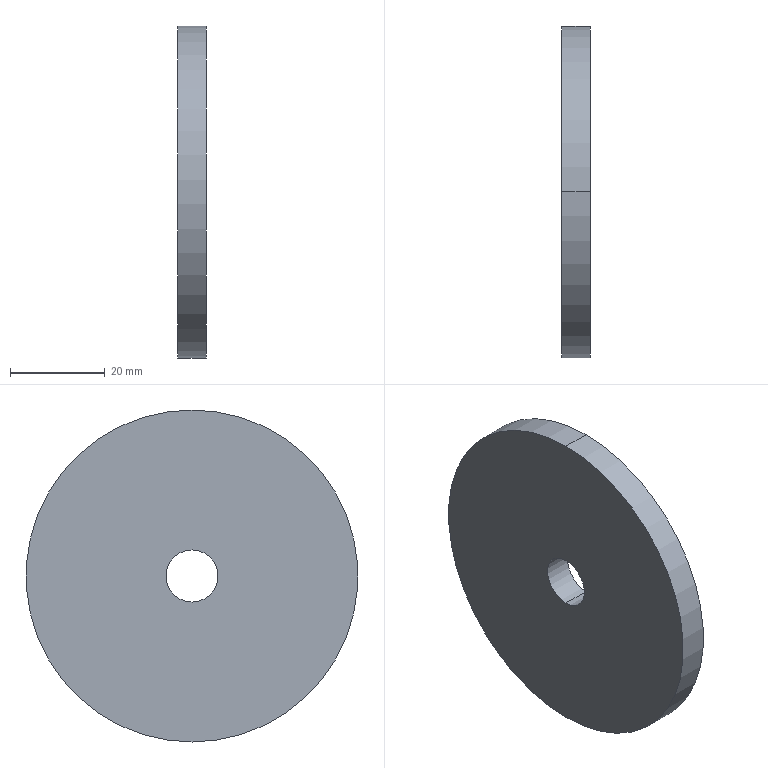Component | SolidWorks | YC1-250-03-01SliderAssembly-1_YC1-250-03-37Gland-1 | 1 solid | 6 faces | box 6 x 70 x 70 mm | volume 22521 mm3 | cylinder 4 | plane 2 | commonest cylinder face diameters 70 x2 11 x2 | material Plain Carbon Steel
STEP:
#1=CARTESIAN_POINT('',(-14.331,110.632,-1.378));
#2=VERTEX_POINT('',#1);
#3=CARTESIAN_POINT('',(-14.331,110.632,1.378));
#4=VERTEX_POINT('',#3);
#5=CARTESIAN_POINT('',(-14.331,110.632,-0.));
#6=DIRECTION('',(1.,0.,0.));
#7=DIRECTION('',(0.,0.,1.));
#8=AXIS2_PLACEMENT_3D('',#5,#6,#7);
#9=CIRCLE('',#8,1.378);
#10=EDGE_CURVE('',#2,#4,#9,.T.);
#11=ORIENTED_EDGE('',*,*,#10,.F.);
#12=CARTESIAN_POINT('',(-14.567,110.632,-1.378));
#13=VERTEX_POINT('',#12);
#14=CARTESIAN_POINT('',(-14.331,110.632,-1.378));
#15=DIRECTION('',(-1.,0.,0.));
#16=VECTOR('',#15,39.37);
#17=LINE('',#14,#16);
#18=EDGE_CURVE('',#2,#13,#17,.T.);
#19=ORIENTED_EDGE('',*,*,#18,.T.);
#20=CARTESIAN_POINT('',(-14.567,110.632,1.378));
#21=VERTEX_POINT('',#20);
#22=CARTESIAN_POINT('',(-14.567,110.632,-0.));
#23=DIRECTION('',(1.,0.,0.));
#24=DIRECTION('',(0.,0.,1.));
#25=AXIS2_PLACEMENT_3D('',#22,#23,#24);
#26=CIRCLE('',#25,1.378);
#27=EDGE_CURVE('',#13,#21,#26,.T.);
#28=ORIENTED_EDGE('',*,*,#27,.T.);
#29=CARTESIAN_POINT('',(-14.331,110.632,1.378));
#30=DIRECTION('',(-1.,0.,0.));
#31=VECTOR('',#30,39.37);
#32=LINE('',#29,#31);
#33=EDGE_CURVE('',#4,#21,#32,.T.);
#34=ORIENTED_EDGE('',*,*,#33,.F.);
#35=EDGE_LOOP('',(#11,#19,#28,#34));
#36=FACE_OUTER_BOUND('',#35,.T.);
#37=CARTESIAN_POINT('',(-14.331,110.632,-0.));
#38=DIRECTION('',(-1.,0.,0.));
#39=DIRECTION('',(0.,0.,1.));
#40=AXIS2_PLACEMENT_3D('',#37,#38,#39);
#41=CYLINDRICAL_SURFACE('',#40,1.378);
#42=ADVANCED_FACE('',(#36),#41,.T.);
#43=CARTESIAN_POINT('',(-14.567,110.632,0.2165));
#44=VERTEX_POINT('',#43);
#45=CARTESIAN_POINT('',(-14.567,110.632,-0.2165));
#46=VERTEX_POINT('',#45);
#47=CARTESIAN_POINT('',(-14.567,110.632,-0.));
#48=DIRECTION('',(1.,0.,0.));
#49=DIRECTION('',(0.,0.,-1.));
#50=AXIS2_PLACEMENT_3D('',#47,#48,#49);
#51=CIRCLE('',#50,0.2165);
#52=EDGE_CURVE('',#44,#46,#51,.T.);
#53=ORIENTED_EDGE('',*,*,#52,.F.);
#54=CARTESIAN_POINT('',(-14.331,110.632,0.2165));
#55=VERTEX_POINT('',#54);
#56=CARTESIAN_POINT('',(-14.331,110.632,0.2165));
#57=DIRECTION('',(1.,0.,0.));
#58=VECTOR('',#57,39.37);
#59=LINE('',#56,#58);
#60=EDGE_CURVE('',#44,#55,#59,.T.);
#61=ORIENTED_EDGE('',*,*,#60,.T.);
#62=CARTESIAN_POINT('',(-14.331,110.632,-0.2165));
#63=VERTEX_POINT('',#62);
#64=CARTESIAN_POINT('',(-14.331,110.632,-0.));
#65=DIRECTION('',(-1.,0.,0.));
#66=DIRECTION('',(0.,0.,-1.));
#67=AXIS2_PLACEMENT_3D('',#64,#65,#66);
#68=CIRCLE('',#67,0.2165);
#69=EDGE_CURVE('',#63,#55,#68,.T.);
#70=ORIENTED_EDGE('',*,*,#69,.F.);
#71=CARTESIAN_POINT('',(-14.331,110.632,-0.2165));
#72=DIRECTION('',(1.,0.,0.));
#73=VECTOR('',#72,39.37);
#74=LINE('',#71,#73);
#75=EDGE_CURVE('',#46,#63,#74,.T.);
#76=ORIENTED_EDGE('',*,*,#75,.F.);
#77=EDGE_LOOP('',(#53,#61,#70,#76));
#78=FACE_OUTER_BOUND('',#77,.T.);
#79=CARTESIAN_POINT('',(-14.331,110.632,-0.));
#80=DIRECTION('',(1.,0.,0.));
#81=DIRECTION('',(0.,0.,-1.));
#82=AXIS2_PLACEMENT_3D('',#79,#80,#81);
#83=CYLINDRICAL_SURFACE('',#82,0.2165);
#84=ADVANCED_FACE('',(#78),#83,.F.);
#85=CARTESIAN_POINT('',(-14.331,110.632,-0.));
#86=DIRECTION('',(1.,0.,0.));
#87=DIRECTION('',(0.,0.,1.));
#88=AXIS2_PLACEMENT_3D('',#85,#86,#87);
#89=CIRCLE('',#88,1.378);
#90=EDGE_CURVE('',#4,#2,#89,.T.);
#91=ORIENTED_EDGE('',*,*,#90,.T.);
#92=ORIENTED_EDGE('',*,*,#10,.T.);
#93=EDGE_LOOP('',(#91,#92));
#94=FACE_OUTER_BOUND('',#93,.T.);
#95=ORIENTED_EDGE('',*,*,#69,.T.);
#96=CARTESIAN_POINT('',(-14.331,110.632,-0.));
#97=DIRECTION('',(-1.,0.,0.));
#98=DIRECTION('',(0.,0.,-1.));
#99=AXIS2_PLACEMENT_3D('',#96,#97,#98);
#100=CIRCLE('',#99,0.2165);
#101=EDGE_CURVE('',#55,#63,#100,.T.);
#102=ORIENTED_EDGE('',*,*,#101,.T.);
#103=EDGE_LOOP('',(#95,#102));
#104=FACE_BOUND('',#103,.T.);
#105=CARTESIAN_POINT('',(-14.331,110.632,-0.));
#106=DIRECTION('',(1.,0.,0.));
#107=DIRECTION('',(0.,0.,-1.));
#108=AXIS2_PLACEMENT_3D('',#105,#106,#107);
#109=PLANE('',#108);
#110=ADVANCED_FACE('',(#94,#104),#109,.T.);
#111=ORIENTED_EDGE('',*,*,#18,.F.);
#112=ORIENTED_EDGE('',*,*,#90,.F.);
#113=ORIENTED_EDGE('',*,*,#33,.T.);
#114=CARTESIAN_POINT('',(-14.567,110.632,-0.));
#115=DIRECTION('',(1.,0.,0.));
#116=DIRECTION('',(0.,0.,1.));
#117=AXIS2_PLACEMENT_3D('',#114,#115,#116);
#118=CIRCLE('',#117,1.378);
#119=EDGE_CURVE('',#21,#13,#118,.T.);
#120=ORIENTED_EDGE('',*,*,#119,.T.);
#121=EDGE_LOOP('',(#111,#112,#113,#120));
#122=FACE_OUTER_BOUND('',#121,.T.);
#123=CARTESIAN_POINT('',(-14.331,110.632,-0.));
#124=DIRECTION('',(-1.,0.,0.));
#125=DIRECTION('',(0.,0.,1.));
#126=AXIS2_PLACEMENT_3D('',#123,#124,#125);
#127=CYLINDRICAL_SURFACE('',#126,1.378);
#128=ADVANCED_FACE('',(#122),#127,.T.);
#129=ORIENTED_EDGE('',*,*,#60,.F.);
#130=CARTESIAN_POINT('',(-14.567,110.632,-0.));
#131=DIRECTION('',(1.,0.,0.));
#132=DIRECTION('',(0.,0.,-1.));
#133=AXIS2_PLACEMENT_3D('',#130,#131,#132);
#134=CIRCLE('',#133,0.2165);
#135=EDGE_CURVE('',#46,#44,#134,.T.);
#136=ORIENTED_EDGE('',*,*,#135,.F.);
#137=ORIENTED_EDGE('',*,*,#75,.T.);
#138=ORIENTED_EDGE('',*,*,#101,.F.);
#139=EDGE_LOOP('',(#129,#136,#137,#138));
#140=FACE_OUTER_BOUND('',#139,.T.);
#141=CARTESIAN_POINT('',(-14.331,110.632,-0.));
#142=DIRECTION('',(1.,0.,0.));
#143=DIRECTION('',(0.,0.,-1.));
#144=AXIS2_PLACEMENT_3D('',#141,#142,#143);
#145=CYLINDRICAL_SURFACE('',#144,0.2165);
#146=ADVANCED_FACE('',(#140),#145,.F.);
#147=ORIENTED_EDGE('',*,*,#119,.F.);
#148=ORIENTED_EDGE('',*,*,#27,.F.);
#149=EDGE_LOOP('',(#147,#148));
#150=FACE_OUTER_BOUND('',#149,.T.);
#151=ORIENTED_EDGE('',*,*,#135,.T.);
#152=ORIENTED_EDGE('',*,*,#52,.T.);
#153=EDGE_LOOP('',(#151,#152));
#154=FACE_BOUND('',#153,.T.);
#155=CARTESIAN_POINT('',(-14.567,110.632,-0.));
#156=DIRECTION('',(1.,0.,0.));
#157=DIRECTION('',(0.,0.,-1.));
#158=AXIS2_PLACEMENT_3D('',#155,#156,#157);
#159=PLANE('',#158);
#160=ADVANCED_FACE('',(#150,#154),#159,.F.);
#161=CLOSED_SHELL('',(#42,#84,#110,#128,#146,#160));
#162=MANIFOLD_SOLID_BREP('',#161);
#163=CARTESIAN_POINT('',(0.,0.,0.));
#164=DIRECTION('',(0.,0.,1.));
#165=DIRECTION('',(1.,0.,0.));
#166=AXIS2_PLACEMENT_3D('',#163,#164,#165);
#167=(LENGTH_UNIT()NAMED_UNIT(*)SI_UNIT($,.METRE.));
#168=LENGTH_MEASURE_WITH_UNIT(LENGTH_MEASURE(0.0254),#167);
#169=DIMENSIONAL_EXPONENTS(1.,0.,0.,0.,0.,0.,0.);
#170=(CONVERSION_BASED_UNIT('',#168)LENGTH_UNIT()NAMED_UNIT(#169));
#171=UNCERTAINTY_MEASURE_WITH_UNIT(LENGTH_MEASURE(0.00001),#170,'','');
#172=(NAMED_UNIT(*)PLANE_ANGLE_UNIT()SI_UNIT($,.RADIAN.));
#173=(NAMED_UNIT(*)SI_UNIT($,.STERADIAN.)SOLID_ANGLE_UNIT());
#174=(GEOMETRIC_REPRESENTATION_CONTEXT(3)GLOBAL_UNCERTAINTY_ASSIGNED_CONTEXT((#171))GLOBAL_UNIT_ASSIGNED_CONTEXT((#170,#172,#173))REPRESENTATION_CONTEXT('',''));
#175=ADVANCED_BREP_SHAPE_REPRESENTATION('',(#162,#166),#174);
#176=COLOUR_RGB('',0.7922,0.8196,0.9333);
#177=FILL_AREA_STYLE_COLOUR('',#176);
#178=FILL_AREA_STYLE('',(#177));
#179=SURFACE_STYLE_FILL_AREA(#178);
#180=SURFACE_SIDE_STYLE('',(#179));
#181=SURFACE_STYLE_USAGE(.BOTH.,#180);
#182=PRESENTATION_STYLE_ASSIGNMENT((#181));
#183=STYLED_ITEM('',(#182),#162);
#184=PRESENTATION_LAYER_ASSIGNMENT('','',(#183));
#185=(LENGTH_UNIT()NAMED_UNIT(*)SI_UNIT($,.METRE.));
#186=LENGTH_MEASURE_WITH_UNIT(LENGTH_MEASURE(0.0254),#185);
#187=DIMENSIONAL_EXPONENTS(1.,0.,0.,0.,0.,0.,0.);
#188=(CONVERSION_BASED_UNIT('',#186)LENGTH_UNIT()NAMED_UNIT(#187));
#189=UNCERTAINTY_MEASURE_WITH_UNIT(LENGTH_MEASURE(0.00001),#188,'','');
#190=(NAMED_UNIT(*)PLANE_ANGLE_UNIT()SI_UNIT($,.RADIAN.));
#191=(NAMED_UNIT(*)SI_UNIT($,.STERADIAN.)SOLID_ANGLE_UNIT());
#192=(GEOMETRIC_REPRESENTATION_CONTEXT(3)GLOBAL_UNCERTAINTY_ASSIGNED_CONTEXT((#189))GLOBAL_UNIT_ASSIGNED_CONTEXT((#188,#190,#191))REPRESENTATION_CONTEXT('',''));
#193=MECHANICAL_DESIGN_GEOMETRIC_PRESENTATION_REPRESENTATION('',(#183),#192);